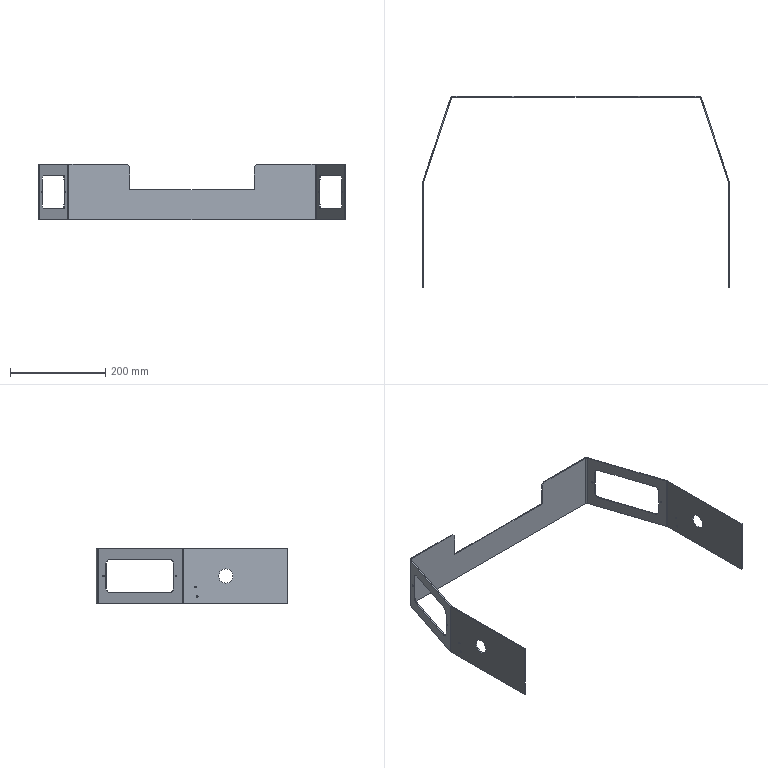Component | SolidWorks | THK-B1016UpperCoverPlate-1 | 1 solid | 80 faces | volume 238984 mm3 | plane 44 | cylinder 36 | commonest cylinder face diameters 3.3 x16 20 x8 30 x4 10 x4 6 x4 | material Q235A